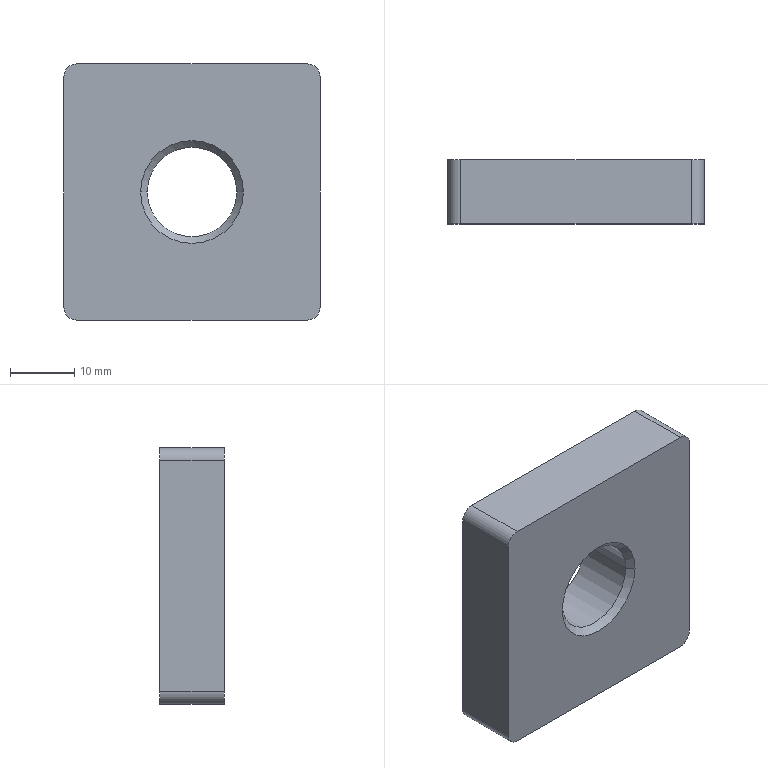Component | SolidWorks | FrameAssembly-1_FrameWeldment-1_AnchorThreadPlate-2 | 1 solid | 14 faces | box 40 x 10 x 40 mm | volume 14402 mm3 | cylinder 6 | plane 6 | cone 2 | commonest cylinder face diameters 4 x4 14 x2
build123d program:
from build123d import *

# Parameters (mm, degrees)
BOSS_EXTRUDE1_DEPTH                                 = 10
CONICAL_COUNTERSUNK_HOLE_1_FOR_M12_FLAT_D           = 14
CONICAL_COUNTERSUNK_HOLE_1_FOR_M12_FLAT_CSINK_D     = 16.05
CONICAL_COUNTERSUNK_HOLE_1_FOR_M12_FLAT_CSINK_ANGLE = 90


with BuildPart() as part:
    # Sketch1 → Boss-Extrude1 (new body)
    with BuildSketch(Plane.XY.offset(5)):
        with BuildLine():
            Line((18, 20), (-18, 20))
            ThreePointArc((-18, 20), (-19.414, 19.414), (-20, 18))
            Line((-20, 18), (-20, -18))
            ThreePointArc((-20, -18), (-19.414, -19.414), (-18, -20))
            Line((-18, -20), (18, -20))
            ThreePointArc((18, -20), (19.414, -19.414), (20, -18))
            Line((20, -18), (20, 18))
            ThreePointArc((20, 18), (19.414, 19.414), (18, 20))
        make_face()
    extrude(amount=-BOSS_EXTRUDE1_DEPTH)

    # Conical Countersunk Hole 1 for M12 Flat (through all)
    with Locations(Plane.XY.offset(5)):
        with Locations((0, 0)):
            CounterSinkHole(CONICAL_COUNTERSUNK_HOLE_1_FOR_M12_FLAT_D / 2, CONICAL_COUNTERSUNK_HOLE_1_FOR_M12_FLAT_CSINK_D / 2, counter_sink_angle=CONICAL_COUNTERSUNK_HOLE_1_FOR_M12_FLAT_CSINK_ANGLE)


solid = part.part

# Placed as in the assembly
solid = solid.moved(Location((-641.246, -443.627, 358.5), (90, 0, 0)))
STEP:
#1=CARTESIAN_POINT('',(-25.522,-17.622,14.114));
#2=VERTEX_POINT('',#1);
#3=CARTESIAN_POINT('',(-24.97,-17.622,14.114));
#4=VERTEX_POINT('',#3);
#5=CARTESIAN_POINT('',(-25.246,-17.622,14.114));
#6=DIRECTION('',(-0.,-1.,0.));
#7=DIRECTION('',(1.,0.,0.));
#8=AXIS2_PLACEMENT_3D('',#5,#6,#7);
#9=CIRCLE('',#8,0.2756);
#10=EDGE_CURVE('',#2,#4,#9,.T.);
#11=ORIENTED_EDGE('',*,*,#10,.F.);
#12=CARTESIAN_POINT('',(-25.562,-17.662,14.114));
#13=VERTEX_POINT('',#12);
#14=CARTESIAN_POINT('',(-25.562,-17.662,14.114));
#15=DIRECTION('',(-0.7071,-0.7071,0.));
#16=VECTOR('',#15,39.37);
#17=LINE('',#14,#16);
#18=EDGE_CURVE('',#2,#13,#17,.T.);
#19=ORIENTED_EDGE('',*,*,#18,.T.);
#20=CARTESIAN_POINT('',(-24.93,-17.662,14.114));
#21=VERTEX_POINT('',#20);
#22=CARTESIAN_POINT('',(-25.246,-17.662,14.114));
#23=DIRECTION('',(-0.,-1.,0.));
#24=DIRECTION('',(1.,0.,0.));
#25=AXIS2_PLACEMENT_3D('',#22,#23,#24);
#26=CIRCLE('',#25,0.3159);
#27=EDGE_CURVE('',#13,#21,#26,.T.);
#28=ORIENTED_EDGE('',*,*,#27,.T.);
#29=CARTESIAN_POINT('',(-24.93,-17.662,14.114));
#30=DIRECTION('',(0.7071,-0.7071,-0.));
#31=VECTOR('',#30,39.37);
#32=LINE('',#29,#31);
#33=EDGE_CURVE('',#4,#21,#32,.T.);
#34=ORIENTED_EDGE('',*,*,#33,.F.);
#35=EDGE_LOOP('',(#11,#19,#28,#34));
#36=FACE_OUTER_BOUND('',#35,.T.);
#37=CARTESIAN_POINT('',(-25.246,-17.662,14.114));
#38=DIRECTION('',(-0.,-1.,0.));
#39=DIRECTION('',(1.,0.,0.));
#40=AXIS2_PLACEMENT_3D('',#37,#38,#39);
#41=CONICAL_SURFACE('',#40,0.3159,0.7854);
#42=ADVANCED_FACE('',(#36),#41,.F.);
#43=CARTESIAN_POINT('',(-25.522,-17.269,14.114));
#44=VERTEX_POINT('',#43);
#45=CARTESIAN_POINT('',(-24.97,-17.269,14.114));
#46=VERTEX_POINT('',#45);
#47=CARTESIAN_POINT('',(-25.246,-17.269,14.114));
#48=DIRECTION('',(-0.,-1.,0.));
#49=DIRECTION('',(1.,0.,0.));
#50=AXIS2_PLACEMENT_3D('',#47,#48,#49);
#51=CIRCLE('',#50,0.2756);
#52=EDGE_CURVE('',#44,#46,#51,.T.);
#53=ORIENTED_EDGE('',*,*,#52,.F.);
#54=CARTESIAN_POINT('',(-25.522,-17.662,14.114));
#55=DIRECTION('',(-0.,-1.,0.));
#56=VECTOR('',#55,39.37);
#57=LINE('',#54,#56);
#58=EDGE_CURVE('',#44,#2,#57,.T.);
#59=ORIENTED_EDGE('',*,*,#58,.T.);
#60=ORIENTED_EDGE('',*,*,#10,.T.);
#61=CARTESIAN_POINT('',(-24.97,-17.662,14.114));
#62=DIRECTION('',(-0.,-1.,0.));
#63=VECTOR('',#62,39.37);
#64=LINE('',#61,#63);
#65=EDGE_CURVE('',#46,#4,#64,.T.);
#66=ORIENTED_EDGE('',*,*,#65,.F.);
#67=EDGE_LOOP('',(#53,#59,#60,#66));
#68=FACE_OUTER_BOUND('',#67,.T.);
#69=CARTESIAN_POINT('',(-25.246,-17.662,14.114));
#70=DIRECTION('',(-0.,-1.,0.));
#71=DIRECTION('',(1.,0.,0.));
#72=AXIS2_PLACEMENT_3D('',#69,#70,#71);
#73=CYLINDRICAL_SURFACE('',#72,0.2756);
#74=ADVANCED_FACE('',(#68),#73,.F.);
#75=CARTESIAN_POINT('',(-24.459,-17.662,14.823));
#76=VERTEX_POINT('',#75);
#77=CARTESIAN_POINT('',(-24.537,-17.662,14.902));
#78=VERTEX_POINT('',#77);
#79=CARTESIAN_POINT('',(-24.537,-17.662,14.823));
#80=DIRECTION('',(-0.,-1.,0.));
#81=DIRECTION('',(1.,0.,0.));
#82=AXIS2_PLACEMENT_3D('',#79,#80,#81);
#83=CIRCLE('',#82,0.07874);
#84=EDGE_CURVE('',#76,#78,#83,.T.);
#85=ORIENTED_EDGE('',*,*,#84,.F.);
#86=CARTESIAN_POINT('',(-24.459,-17.269,14.823));
#87=VERTEX_POINT('',#86);
#88=CARTESIAN_POINT('',(-24.459,-17.269,14.823));
#89=DIRECTION('',(-0.,-1.,0.));
#90=VECTOR('',#89,39.37);
#91=LINE('',#88,#90);
#92=EDGE_CURVE('',#87,#76,#91,.T.);
#93=ORIENTED_EDGE('',*,*,#92,.F.);
#94=CARTESIAN_POINT('',(-24.537,-17.269,14.902));
#95=VERTEX_POINT('',#94);
#96=CARTESIAN_POINT('',(-24.537,-17.269,14.823));
#97=DIRECTION('',(-0.,-1.,0.));
#98=DIRECTION('',(1.,0.,0.));
#99=AXIS2_PLACEMENT_3D('',#96,#97,#98);
#100=CIRCLE('',#99,0.07874);
#101=EDGE_CURVE('',#87,#95,#100,.T.);
#102=ORIENTED_EDGE('',*,*,#101,.T.);
#103=CARTESIAN_POINT('',(-24.537,-17.269,14.902));
#104=DIRECTION('',(-0.,-1.,0.));
#105=VECTOR('',#104,39.37);
#106=LINE('',#103,#105);
#107=EDGE_CURVE('',#95,#78,#106,.T.);
#108=ORIENTED_EDGE('',*,*,#107,.T.);
#109=EDGE_LOOP('',(#85,#93,#102,#108));
#110=FACE_OUTER_BOUND('',#109,.T.);
#111=CARTESIAN_POINT('',(-24.537,-17.269,14.823));
#112=DIRECTION('',(-0.,-1.,0.));
#113=DIRECTION('',(1.,0.,0.));
#114=AXIS2_PLACEMENT_3D('',#111,#112,#113);
#115=CYLINDRICAL_SURFACE('',#114,0.07874);
#116=ADVANCED_FACE('',(#110),#115,.T.);
#117=CARTESIAN_POINT('',(-24.459,-17.662,13.406));
#118=VERTEX_POINT('',#117);
#119=CARTESIAN_POINT('',(-24.459,-17.662,13.406));
#120=DIRECTION('',(0.,0.,1.));
#121=VECTOR('',#120,39.37);
#122=LINE('',#119,#121);
#123=EDGE_CURVE('',#118,#76,#122,.T.);
#124=ORIENTED_EDGE('',*,*,#123,.F.);
#125=CARTESIAN_POINT('',(-24.459,-17.269,13.406));
#126=VERTEX_POINT('',#125);
#127=CARTESIAN_POINT('',(-24.459,-17.269,13.406));
#128=DIRECTION('',(-0.,-1.,0.));
#129=VECTOR('',#128,39.37);
#130=LINE('',#127,#129);
#131=EDGE_CURVE('',#126,#118,#130,.T.);
#132=ORIENTED_EDGE('',*,*,#131,.F.);
#133=CARTESIAN_POINT('',(-24.459,-17.269,13.406));
#134=DIRECTION('',(0.,0.,1.));
#135=VECTOR('',#134,39.37);
#136=LINE('',#133,#135);
#137=EDGE_CURVE('',#126,#87,#136,.T.);
#138=ORIENTED_EDGE('',*,*,#137,.T.);
#139=ORIENTED_EDGE('',*,*,#92,.T.);
#140=EDGE_LOOP('',(#124,#132,#138,#139));
#141=FACE_OUTER_BOUND('',#140,.T.);
#142=CARTESIAN_POINT('',(-24.459,-17.269,13.406));
#143=DIRECTION('',(1.,-0.,-0.));
#144=DIRECTION('',(0.,0.,1.));
#145=AXIS2_PLACEMENT_3D('',#142,#143,#144);
#146=PLANE('',#145);
#147=ADVANCED_FACE('',(#141),#146,.T.);
#148=CARTESIAN_POINT('',(-24.537,-17.662,13.327));
#149=VERTEX_POINT('',#148);
#150=CARTESIAN_POINT('',(-24.537,-17.662,13.406));
#151=DIRECTION('',(-0.,-1.,0.));
#152=DIRECTION('',(1.,0.,0.));
#153=AXIS2_PLACEMENT_3D('',#150,#151,#152);
#154=CIRCLE('',#153,0.07874);
#155=EDGE_CURVE('',#149,#118,#154,.T.);
#156=ORIENTED_EDGE('',*,*,#155,.F.);
#157=CARTESIAN_POINT('',(-24.537,-17.269,13.327));
#158=VERTEX_POINT('',#157);
#159=CARTESIAN_POINT('',(-24.537,-17.269,13.327));
#160=DIRECTION('',(-0.,-1.,0.));
#161=VECTOR('',#160,39.37);
#162=LINE('',#159,#161);
#163=EDGE_CURVE('',#158,#149,#162,.T.);
#164=ORIENTED_EDGE('',*,*,#163,.F.);
#165=CARTESIAN_POINT('',(-24.537,-17.269,13.406));
#166=DIRECTION('',(-0.,-1.,0.));
#167=DIRECTION('',(1.,0.,0.));
#168=AXIS2_PLACEMENT_3D('',#165,#166,#167);
#169=CIRCLE('',#168,0.07874);
#170=EDGE_CURVE('',#158,#126,#169,.T.);
#171=ORIENTED_EDGE('',*,*,#170,.T.);
#172=ORIENTED_EDGE('',*,*,#131,.T.);
#173=EDGE_LOOP('',(#156,#164,#171,#172));
#174=FACE_OUTER_BOUND('',#173,.T.);
#175=CARTESIAN_POINT('',(-24.537,-17.269,13.406));
#176=DIRECTION('',(-0.,-1.,0.));
#177=DIRECTION('',(1.,0.,0.));
#178=AXIS2_PLACEMENT_3D('',#175,#176,#177);
#179=CYLINDRICAL_SURFACE('',#178,0.07874);
#180=ADVANCED_FACE('',(#174),#179,.T.);
#181=CARTESIAN_POINT('',(-25.955,-17.662,13.327));
#182=VERTEX_POINT('',#181);
#183=CARTESIAN_POINT('',(-25.955,-17.662,13.327));
#184=DIRECTION('',(1.,-0.,-0.));
#185=VECTOR('',#184,39.37);
#186=LINE('',#183,#185);
#187=EDGE_CURVE('',#182,#149,#186,.T.);
#188=ORIENTED_EDGE('',*,*,#187,.F.);
#189=CARTESIAN_POINT('',(-25.955,-17.269,13.327));
#190=VERTEX_POINT('',#189);
#191=CARTESIAN_POINT('',(-25.955,-17.269,13.327));
#192=DIRECTION('',(-0.,-1.,0.));
#193=VECTOR('',#192,39.37);
#194=LINE('',#191,#193);
#195=EDGE_CURVE('',#190,#182,#194,.T.);
#196=ORIENTED_EDGE('',*,*,#195,.F.);
#197=CARTESIAN_POINT('',(-25.955,-17.269,13.327));
#198=DIRECTION('',(1.,-0.,-0.));
#199=VECTOR('',#198,39.37);
#200=LINE('',#197,#199);
#201=EDGE_CURVE('',#190,#158,#200,.T.);
#202=ORIENTED_EDGE('',*,*,#201,.T.);
#203=ORIENTED_EDGE('',*,*,#163,.T.);
#204=EDGE_LOOP('',(#188,#196,#202,#203));
#205=FACE_OUTER_BOUND('',#204,.T.);
#206=CARTESIAN_POINT('',(-25.955,-17.269,13.327));
#207=DIRECTION('',(-0.,-0.,-1.));
#208=DIRECTION('',(0.,1.,-0.));
#209=AXIS2_PLACEMENT_3D('',#206,#207,#208);
#210=PLANE('',#209);
#211=ADVANCED_FACE('',(#205),#210,.T.);
#212=CARTESIAN_POINT('',(-26.033,-17.662,13.406));
#213=VERTEX_POINT('',#212);
#214=CARTESIAN_POINT('',(-25.955,-17.662,13.406));
#215=DIRECTION('',(-0.,-1.,0.));
#216=DIRECTION('',(1.,0.,0.));
#217=AXIS2_PLACEMENT_3D('',#214,#215,#216);
#218=CIRCLE('',#217,0.07874);
#219=EDGE_CURVE('',#213,#182,#218,.T.);
#220=ORIENTED_EDGE('',*,*,#219,.F.);
#221=CARTESIAN_POINT('',(-26.033,-17.269,13.406));
#222=VERTEX_POINT('',#221);
#223=CARTESIAN_POINT('',(-26.033,-17.269,13.406));
#224=DIRECTION('',(-0.,-1.,0.));
#225=VECTOR('',#224,39.37);
#226=LINE('',#223,#225);
#227=EDGE_CURVE('',#222,#213,#226,.T.);
#228=ORIENTED_EDGE('',*,*,#227,.F.);
#229=CARTESIAN_POINT('',(-25.955,-17.269,13.406));
#230=DIRECTION('',(-0.,-1.,0.));
#231=DIRECTION('',(1.,0.,0.));
#232=AXIS2_PLACEMENT_3D('',#229,#230,#231);
#233=CIRCLE('',#232,0.07874);
#234=EDGE_CURVE('',#222,#190,#233,.T.);
#235=ORIENTED_EDGE('',*,*,#234,.T.);
#236=ORIENTED_EDGE('',*,*,#195,.T.);
#237=EDGE_LOOP('',(#220,#228,#235,#236));
#238=FACE_OUTER_BOUND('',#237,.T.);
#239=CARTESIAN_POINT('',(-25.955,-17.269,13.406));
#240=DIRECTION('',(-0.,-1.,0.));
#241=DIRECTION('',(1.,0.,0.));
#242=AXIS2_PLACEMENT_3D('',#239,#240,#241);
#243=CYLINDRICAL_SURFACE('',#242,0.07874);
#244=ADVANCED_FACE('',(#238),#243,.T.);
#245=CARTESIAN_POINT('',(-26.033,-17.662,14.823));
#246=VERTEX_POINT('',#245);
#247=CARTESIAN_POINT('',(-26.033,-17.662,14.823));
#248=DIRECTION('',(-0.,-0.,-1.));
#249=VECTOR('',#248,39.37);
#250=LINE('',#247,#249);
#251=EDGE_CURVE('',#246,#213,#250,.T.);
#252=ORIENTED_EDGE('',*,*,#251,.F.);
#253=CARTESIAN_POINT('',(-26.033,-17.269,14.823));
#254=VERTEX_POINT('',#253);
#255=CARTESIAN_POINT('',(-26.033,-17.269,14.823));
#256=DIRECTION('',(-0.,-1.,0.));
#257=VECTOR('',#256,39.37);
#258=LINE('',#255,#257);
#259=EDGE_CURVE('',#254,#246,#258,.T.);
#260=ORIENTED_EDGE('',*,*,#259,.F.);
#261=CARTESIAN_POINT('',(-26.033,-17.269,14.823));
#262=DIRECTION('',(-0.,-0.,-1.));
#263=VECTOR('',#262,39.37);
#264=LINE('',#261,#263);
#265=EDGE_CURVE('',#254,#222,#264,.T.);
#266=ORIENTED_EDGE('',*,*,#265,.T.);
#267=ORIENTED_EDGE('',*,*,#227,.T.);
#268=EDGE_LOOP('',(#252,#260,#266,#267));
#269=FACE_OUTER_BOUND('',#268,.T.);
#270=CARTESIAN_POINT('',(-26.033,-17.269,14.823));
#271=DIRECTION('',(-1.,0.,0.));
#272=DIRECTION('',(-0.,-1.,0.));
#273=AXIS2_PLACEMENT_3D('',#270,#271,#272);
#274=PLANE('',#273);
#275=ADVANCED_FACE('',(#269),#274,.T.);
#276=CARTESIAN_POINT('',(-25.955,-17.662,14.902));
#277=VERTEX_POINT('',#276);
#278=CARTESIAN_POINT('',(-25.955,-17.662,14.823));
#279=DIRECTION('',(-0.,-1.,0.));
#280=DIRECTION('',(1.,0.,0.));
#281=AXIS2_PLACEMENT_3D('',#278,#279,#280);
#282=CIRCLE('',#281,0.07874);
#283=EDGE_CURVE('',#277,#246,#282,.T.);
#284=ORIENTED_EDGE('',*,*,#283,.F.);
#285=CARTESIAN_POINT('',(-25.955,-17.269,14.902));
#286=VERTEX_POINT('',#285);
#287=CARTESIAN_POINT('',(-25.955,-17.269,14.902));
#288=DIRECTION('',(-0.,-1.,0.));
#289=VECTOR('',#288,39.37);
#290=LINE('',#287,#289);
#291=EDGE_CURVE('',#286,#277,#290,.T.);
#292=ORIENTED_EDGE('',*,*,#291,.F.);
#293=CARTESIAN_POINT('',(-25.955,-17.269,14.823));
#294=DIRECTION('',(-0.,-1.,0.));
#295=DIRECTION('',(1.,0.,0.));
#296=AXIS2_PLACEMENT_3D('',#293,#294,#295);
#297=CIRCLE('',#296,0.07874);
#298=EDGE_CURVE('',#286,#254,#297,.T.);
#299=ORIENTED_EDGE('',*,*,#298,.T.);
#300=ORIENTED_EDGE('',*,*,#259,.T.);
#301=EDGE_LOOP('',(#284,#292,#299,#300));
#302=FACE_OUTER_BOUND('',#301,.T.);
#303=CARTESIAN_POINT('',(-25.955,-17.269,14.823));
#304=DIRECTION('',(-0.,-1.,0.));
#305=DIRECTION('',(1.,0.,0.));
#306=AXIS2_PLACEMENT_3D('',#303,#304,#305);
#307=CYLINDRICAL_SURFACE('',#306,0.07874);
#308=ADVANCED_FACE('',(#302),#307,.T.);
#309=CARTESIAN_POINT('',(-24.537,-17.662,14.902));
#310=DIRECTION('',(-1.,0.,0.));
#311=VECTOR('',#310,39.37);
#312=LINE('',#309,#311);
#313=EDGE_CURVE('',#78,#277,#312,.T.);
#314=ORIENTED_EDGE('',*,*,#313,.F.);
#315=ORIENTED_EDGE('',*,*,#107,.F.);
#316=CARTESIAN_POINT('',(-24.537,-17.269,14.902));
#317=DIRECTION('',(-1.,0.,0.));
#318=VECTOR('',#317,39.37);
#319=LINE('',#316,#318);
#320=EDGE_CURVE('',#95,#286,#319,.T.);
#321=ORIENTED_EDGE('',*,*,#320,.T.);
#322=ORIENTED_EDGE('',*,*,#291,.T.);
#323=EDGE_LOOP('',(#314,#315,#321,#322));
#324=FACE_OUTER_BOUND('',#323,.T.);
#325=CARTESIAN_POINT('',(-24.537,-17.269,14.902));
#326=DIRECTION('',(0.,0.,1.));
#327=DIRECTION('',(-0.,-1.,0.));
#328=AXIS2_PLACEMENT_3D('',#325,#326,#327);
#329=PLANE('',#328);
#330=ADVANCED_FACE('',(#324),#329,.T.);
#331=CARTESIAN_POINT('',(-25.246,-17.269,14.114));
#332=DIRECTION('',(-0.,-1.,0.));
#333=DIRECTION('',(1.,0.,0.));
#334=AXIS2_PLACEMENT_3D('',#331,#332,#333);
#335=CIRCLE('',#334,0.2756);
#336=EDGE_CURVE('',#46,#44,#335,.T.);
#337=ORIENTED_EDGE('',*,*,#336,.T.);
#338=ORIENTED_EDGE('',*,*,#52,.T.);
#339=EDGE_LOOP('',(#337,#338));
#340=FACE_BOUND('',#339,.T.);
#341=ORIENTED_EDGE('',*,*,#101,.F.);
#342=ORIENTED_EDGE('',*,*,#137,.F.);
#343=ORIENTED_EDGE('',*,*,#170,.F.);
#344=ORIENTED_EDGE('',*,*,#201,.F.);
#345=ORIENTED_EDGE('',*,*,#234,.F.);
#346=ORIENTED_EDGE('',*,*,#265,.F.);
#347=ORIENTED_EDGE('',*,*,#298,.F.);
#348=ORIENTED_EDGE('',*,*,#320,.F.);
#349=EDGE_LOOP('',(#341,#342,#343,#344,#345,#346,#347,#348));
#350=FACE_OUTER_BOUND('',#349,.T.);
#351=CARTESIAN_POINT('',(-24.537,-17.269,14.823));
#352=DIRECTION('',(-0.,-1.,0.));
#353=DIRECTION('',(1.,-0.,-0.));
#354=AXIS2_PLACEMENT_3D('',#351,#352,#353);
#355=PLANE('',#354);
#356=ADVANCED_FACE('',(#340,#350),#355,.F.);
#357=CARTESIAN_POINT('',(-25.246,-17.662,14.114));
#358=DIRECTION('',(-0.,-1.,0.));
#359=DIRECTION('',(1.,0.,0.));
#360=AXIS2_PLACEMENT_3D('',#357,#358,#359);
#361=CIRCLE('',#360,0.3159);
#362=EDGE_CURVE('',#21,#13,#361,.T.);
#363=ORIENTED_EDGE('',*,*,#362,.F.);
#364=ORIENTED_EDGE('',*,*,#27,.F.);
#365=EDGE_LOOP('',(#363,#364));
#366=FACE_BOUND('',#365,.T.);
#367=ORIENTED_EDGE('',*,*,#84,.T.);
#368=ORIENTED_EDGE('',*,*,#313,.T.);
#369=ORIENTED_EDGE('',*,*,#283,.T.);
#370=ORIENTED_EDGE('',*,*,#251,.T.);
#371=ORIENTED_EDGE('',*,*,#219,.T.);
#372=ORIENTED_EDGE('',*,*,#187,.T.);
#373=ORIENTED_EDGE('',*,*,#155,.T.);
#374=ORIENTED_EDGE('',*,*,#123,.T.);
#375=EDGE_LOOP('',(#367,#368,#369,#370,#371,#372,#373,#374));
#376=FACE_OUTER_BOUND('',#375,.T.);
#377=CARTESIAN_POINT('',(-24.537,-17.662,14.823));
#378=DIRECTION('',(-0.,-1.,0.));
#379=DIRECTION('',(1.,-0.,-0.));
#380=AXIS2_PLACEMENT_3D('',#377,#378,#379);
#381=PLANE('',#380);
#382=ADVANCED_FACE('',(#366,#376),#381,.T.);
#383=ORIENTED_EDGE('',*,*,#58,.F.);
#384=ORIENTED_EDGE('',*,*,#336,.F.);
#385=ORIENTED_EDGE('',*,*,#65,.T.);
#386=CARTESIAN_POINT('',(-25.246,-17.622,14.114));
#387=DIRECTION('',(-0.,-1.,0.));
#388=DIRECTION('',(1.,0.,0.));
#389=AXIS2_PLACEMENT_3D('',#386,#387,#388);
#390=CIRCLE('',#389,0.2756);
#391=EDGE_CURVE('',#4,#2,#390,.T.);
#392=ORIENTED_EDGE('',*,*,#391,.T.);
#393=EDGE_LOOP('',(#383,#384,#385,#392));
#394=FACE_OUTER_BOUND('',#393,.T.);
#395=CARTESIAN_POINT('',(-25.246,-17.662,14.114));
#396=DIRECTION('',(-0.,-1.,0.));
#397=DIRECTION('',(1.,0.,0.));
#398=AXIS2_PLACEMENT_3D('',#395,#396,#397);
#399=CYLINDRICAL_SURFACE('',#398,0.2756);
#400=ADVANCED_FACE('',(#394),#399,.F.);
#401=ORIENTED_EDGE('',*,*,#18,.F.);
#402=ORIENTED_EDGE('',*,*,#391,.F.);
#403=ORIENTED_EDGE('',*,*,#33,.T.);
#404=ORIENTED_EDGE('',*,*,#362,.T.);
#405=EDGE_LOOP('',(#401,#402,#403,#404));
#406=FACE_OUTER_BOUND('',#405,.T.);
#407=CARTESIAN_POINT('',(-25.246,-17.662,14.114));
#408=DIRECTION('',(-0.,-1.,0.));
#409=DIRECTION('',(1.,0.,0.));
#410=AXIS2_PLACEMENT_3D('',#407,#408,#409);
#411=CONICAL_SURFACE('',#410,0.3159,0.7854);
#412=ADVANCED_FACE('',(#406),#411,.F.);
#413=CLOSED_SHELL('',(#42,#74,#116,#147,#180,#211,#244,#275,#308,#330,#356,#382,#400,#412));
#414=MANIFOLD_SOLID_BREP('',#413);
#415=CARTESIAN_POINT('',(0.,0.,0.));
#416=DIRECTION('',(0.,0.,1.));
#417=DIRECTION('',(1.,0.,0.));
#418=AXIS2_PLACEMENT_3D('',#415,#416,#417);
#419=(LENGTH_UNIT()NAMED_UNIT(*)SI_UNIT($,.METRE.));
#420=LENGTH_MEASURE_WITH_UNIT(LENGTH_MEASURE(0.0254),#419);
#421=DIMENSIONAL_EXPONENTS(1.,0.,0.,0.,0.,0.,0.);
#422=(CONVERSION_BASED_UNIT('',#420)LENGTH_UNIT()NAMED_UNIT(#421));
#423=UNCERTAINTY_MEASURE_WITH_UNIT(LENGTH_MEASURE(0.00001),#422,'','');
#424=(NAMED_UNIT(*)PLANE_ANGLE_UNIT()SI_UNIT($,.RADIAN.));
#425=(NAMED_UNIT(*)SI_UNIT($,.STERADIAN.)SOLID_ANGLE_UNIT());
#426=(GEOMETRIC_REPRESENTATION_CONTEXT(3)GLOBAL_UNCERTAINTY_ASSIGNED_CONTEXT((#423))GLOBAL_UNIT_ASSIGNED_CONTEXT((#422,#424,#425))REPRESENTATION_CONTEXT('',''));
#427=ADVANCED_BREP_SHAPE_REPRESENTATION('',(#414,#418),#426);
#428=COLOUR_RGB('',0.7922,0.8196,0.9333);
#429=FILL_AREA_STYLE_COLOUR('',#428);
#430=FILL_AREA_STYLE('',(#429));
#431=SURFACE_STYLE_FILL_AREA(#430);
#432=SURFACE_SIDE_STYLE('',(#431));
#433=SURFACE_STYLE_USAGE(.BOTH.,#432);
#434=PRESENTATION_STYLE_ASSIGNMENT((#433));
#435=STYLED_ITEM('',(#434),#414);
#436=PRESENTATION_LAYER_ASSIGNMENT('','',(#435));
#437=(LENGTH_UNIT()NAMED_UNIT(*)SI_UNIT($,.METRE.));
#438=LENGTH_MEASURE_WITH_UNIT(LENGTH_MEASURE(0.0254),#437);
#439=DIMENSIONAL_EXPONENTS(1.,0.,0.,0.,0.,0.,0.);
#440=(CONVERSION_BASED_UNIT('',#438)LENGTH_UNIT()NAMED_UNIT(#439));
#441=UNCERTAINTY_MEASURE_WITH_UNIT(LENGTH_MEASURE(0.00001),#440,'','');
#442=(NAMED_UNIT(*)PLANE_ANGLE_UNIT()SI_UNIT($,.RADIAN.));
#443=(NAMED_UNIT(*)SI_UNIT($,.STERADIAN.)SOLID_ANGLE_UNIT());
#444=(GEOMETRIC_REPRESENTATION_CONTEXT(3)GLOBAL_UNCERTAINTY_ASSIGNED_CONTEXT((#441))GLOBAL_UNIT_ASSIGNED_CONTEXT((#440,#442,#443))REPRESENTATION_CONTEXT('',''));
#445=MECHANICAL_DESIGN_GEOMETRIC_PRESENTATION_REPRESENTATION('',(#435),#444);